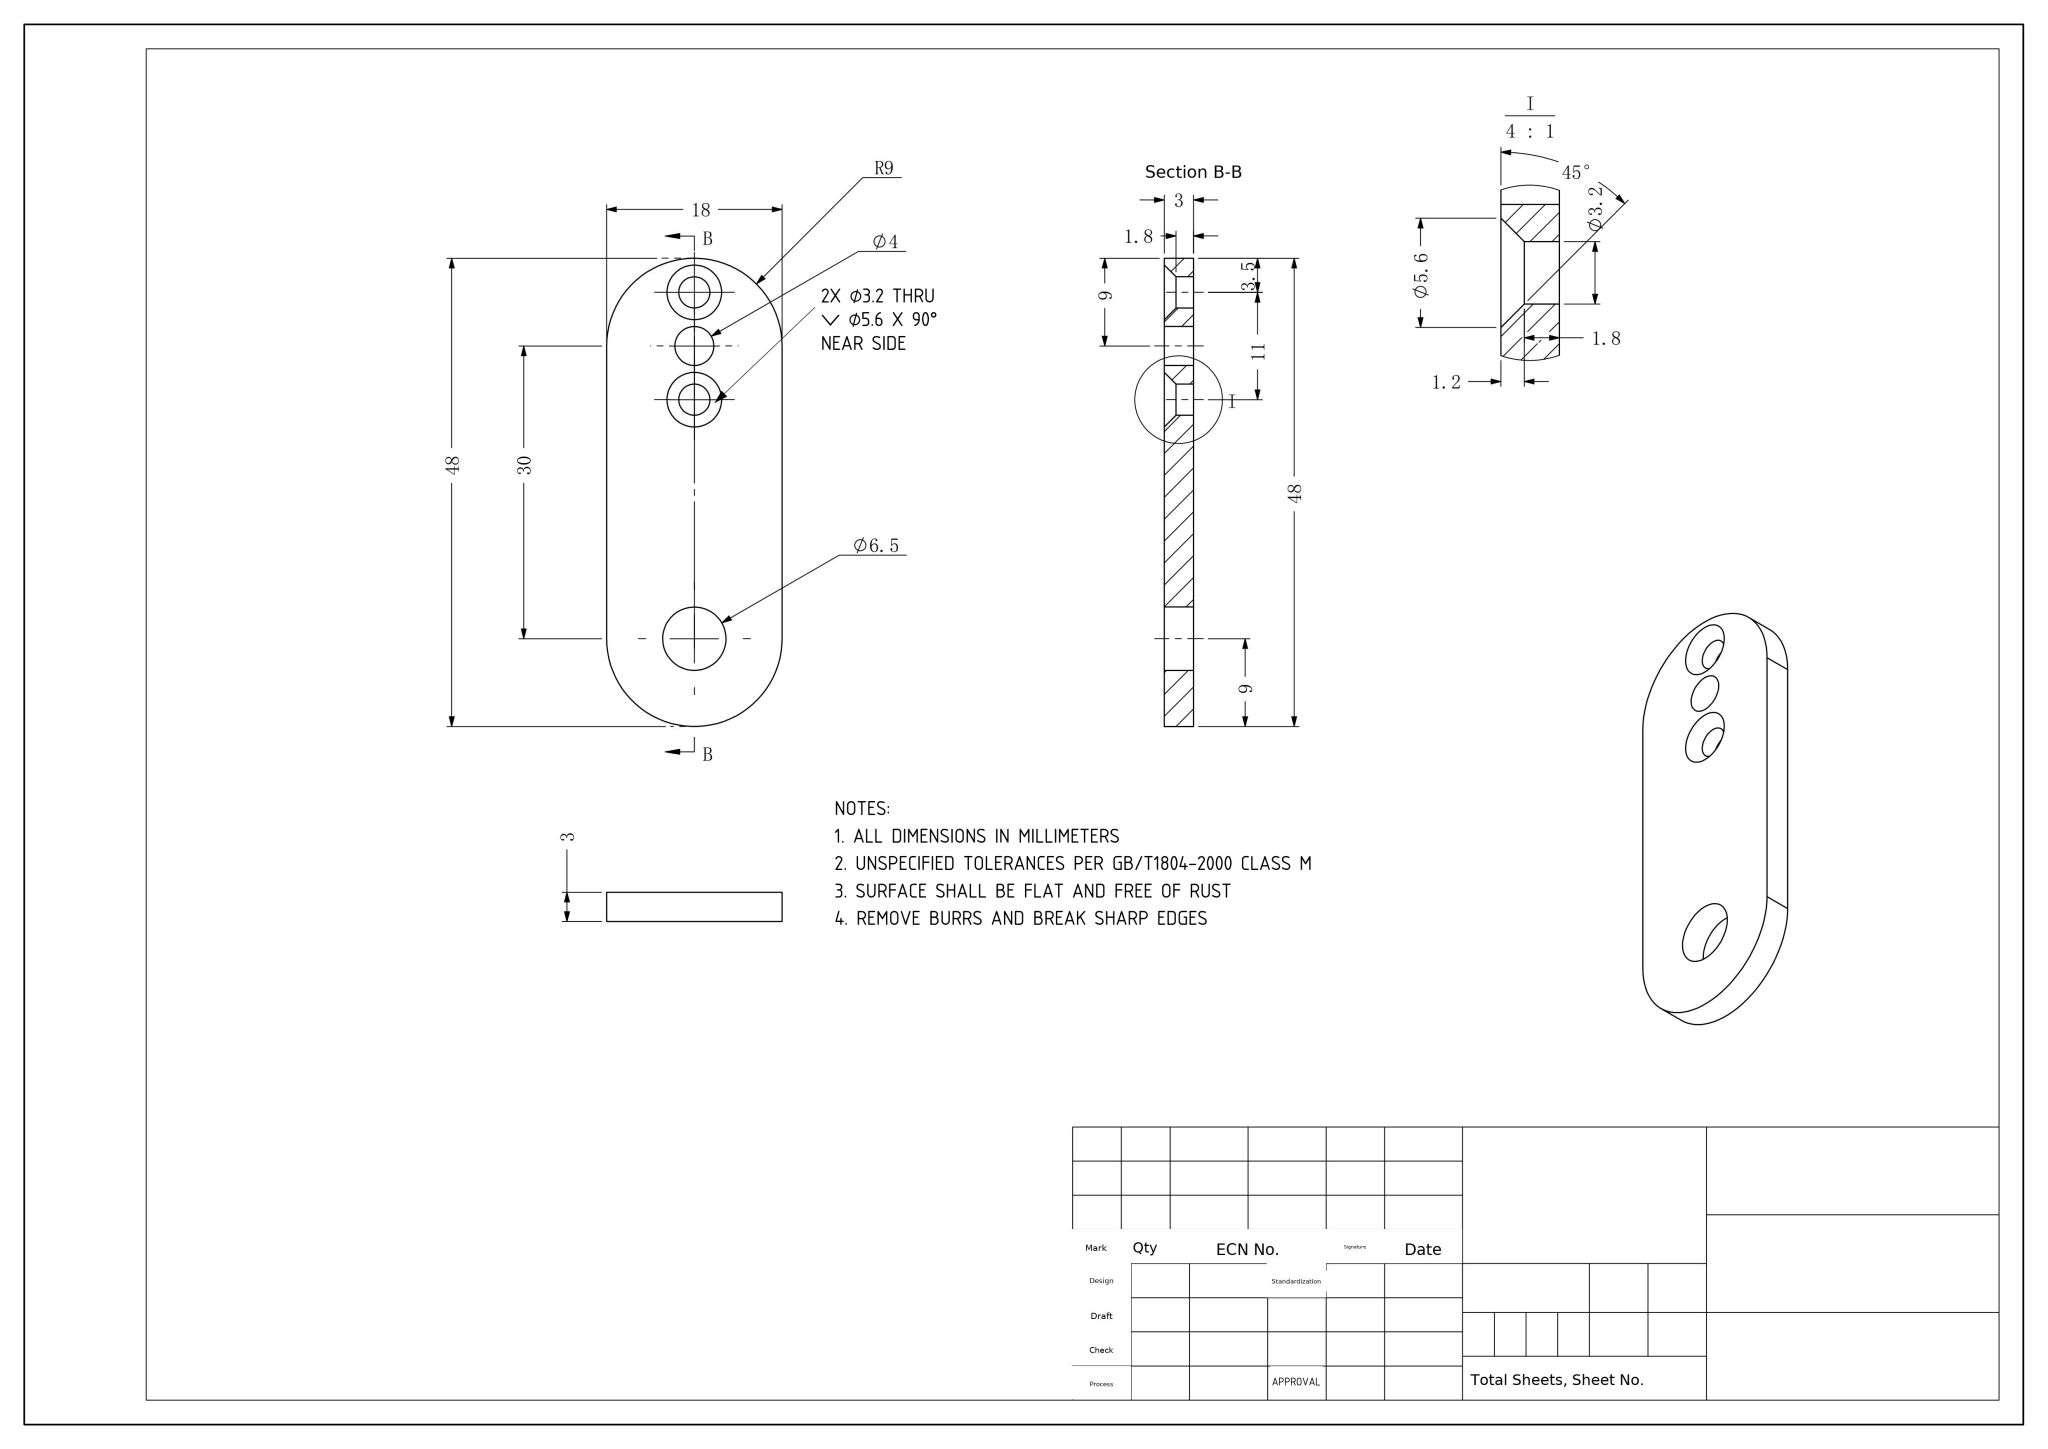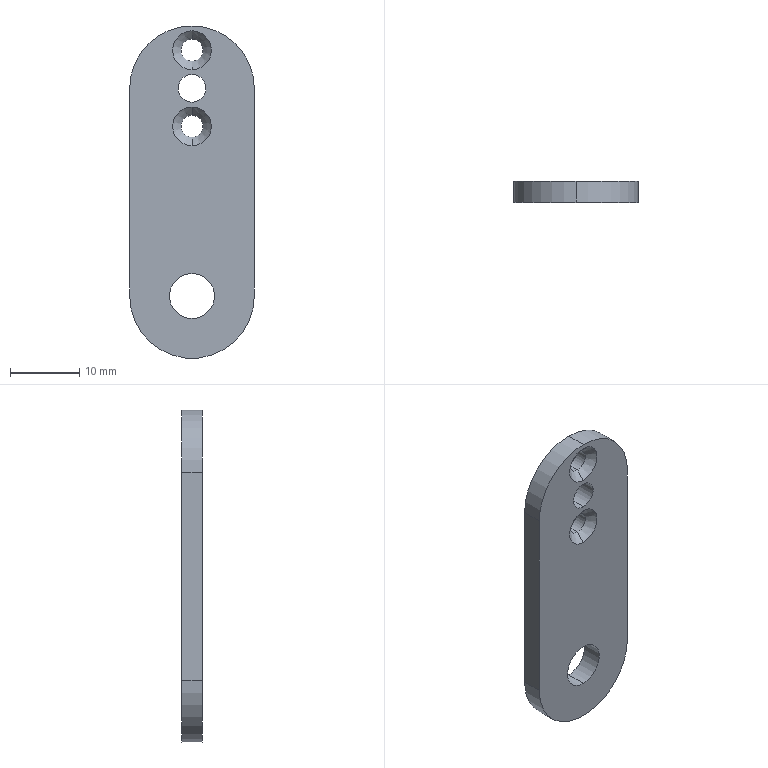Part | NX | mm | Rounded Four-Bore Link Plate | 1 solid | 19 faces | box 18 x 3 x 48 mm | volume 2180 mm3 | cylinder 11 | cone 4 | plane 4 | commonest cylinder face diameters 3.2 x4 18 x3 6.5 x2 4 x2
STEP:
#1=COLOUR_RGB('',0.7529,0.7529,0.7529);
#2=FILL_AREA_STYLE_COLOUR('',#1);
#3=FILL_AREA_STYLE('',(#2));
#4=SURFACE_STYLE_FILL_AREA(#3);
#5=SURFACE_SIDE_STYLE('',(#4));
#6=SURFACE_STYLE_USAGE(.BOTH.,#5);
#7=PRESENTATION_STYLE_ASSIGNMENT((#6));
#8=CARTESIAN_POINT('',(1.,-0.3,21.1));
#9=VERTEX_POINT('',#8);
#10=CARTESIAN_POINT('',(1.,-0.3,17.9));
#11=VERTEX_POINT('',#10);
#12=CARTESIAN_POINT('',(1.,-0.3,19.5));
#13=DIRECTION('',(0.,-1.,0.));
#14=DIRECTION('',(0.,0.,-1.));
#15=AXIS2_PLACEMENT_3D('',#12,#13,#14);
#16=CIRCLE('',#15,1.6);
#17=EDGE_CURVE('',#9,#11,#16,.T.);
#18=ORIENTED_EDGE('',*,*,#17,.F.);
#19=CARTESIAN_POINT('',(1.,-1.5,22.3));
#20=VERTEX_POINT('',#19);
#21=CARTESIAN_POINT('',(1.,-1.5,22.3));
#22=DIRECTION('',(0.,-0.7071,0.7071));
#23=VECTOR('',#22,1000.);
#24=LINE('',#21,#23);
#25=EDGE_CURVE('',#9,#20,#24,.T.);
#26=ORIENTED_EDGE('',*,*,#25,.T.);
#27=CARTESIAN_POINT('',(1.,-1.5,16.7));
#28=VERTEX_POINT('',#27);
#29=CARTESIAN_POINT('',(1.,-1.5,19.5));
#30=DIRECTION('',(0.,1.,0.));
#31=DIRECTION('',(0.,0.,-1.));
#32=AXIS2_PLACEMENT_3D('',#29,#30,#31);
#33=CIRCLE('',#32,2.8);
#34=EDGE_CURVE('',#28,#20,#33,.T.);
#35=ORIENTED_EDGE('',*,*,#34,.F.);
#36=CARTESIAN_POINT('',(1.,-1.5,16.7));
#37=DIRECTION('',(0.,-0.7071,-0.7071));
#38=VECTOR('',#37,1000.);
#39=LINE('',#36,#38);
#40=EDGE_CURVE('',#11,#28,#39,.T.);
#41=ORIENTED_EDGE('',*,*,#40,.F.);
#42=EDGE_LOOP('',(#18,#26,#35,#41));
#43=FACE_OUTER_BOUND('',#42,.T.);
#44=CARTESIAN_POINT('',(1.,-1.5,19.5));
#45=DIRECTION('',(0.,-1.,0.));
#46=DIRECTION('',(0.,0.,-1.));
#47=AXIS2_PLACEMENT_3D('',#44,#45,#46);
#48=CONICAL_SURFACE('',#47,2.8,0.7854);
#49=ADVANCED_FACE('',(#43),#48,.F.);
#50=CARTESIAN_POINT('',(1.,-0.3,10.1));
#51=VERTEX_POINT('',#50);
#52=CARTESIAN_POINT('',(1.,-0.3,6.9));
#53=VERTEX_POINT('',#52);
#54=CARTESIAN_POINT('',(1.,-0.3,8.5));
#55=DIRECTION('',(0.,-1.,0.));
#56=DIRECTION('',(0.,0.,-1.));
#57=AXIS2_PLACEMENT_3D('',#54,#55,#56);
#58=CIRCLE('',#57,1.6);
#59=EDGE_CURVE('',#51,#53,#58,.T.);
#60=ORIENTED_EDGE('',*,*,#59,.F.);
#61=CARTESIAN_POINT('',(1.,-1.5,11.3));
#62=VERTEX_POINT('',#61);
#63=CARTESIAN_POINT('',(1.,-0.3,10.1));
#64=DIRECTION('',(0.,-0.7071,0.7071));
#65=VECTOR('',#64,1000.);
#66=LINE('',#63,#65);
#67=EDGE_CURVE('',#51,#62,#66,.T.);
#68=ORIENTED_EDGE('',*,*,#67,.T.);
#69=CARTESIAN_POINT('',(1.,-1.5,5.7));
#70=VERTEX_POINT('',#69);
#71=CARTESIAN_POINT('',(1.,-1.5,8.5));
#72=DIRECTION('',(0.,1.,0.));
#73=DIRECTION('',(0.,0.,-1.));
#74=AXIS2_PLACEMENT_3D('',#71,#72,#73);
#75=CIRCLE('',#74,2.8);
#76=EDGE_CURVE('',#70,#62,#75,.T.);
#77=ORIENTED_EDGE('',*,*,#76,.F.);
#78=CARTESIAN_POINT('',(1.,-0.3,6.9));
#79=DIRECTION('',(0.,-0.7071,-0.7071));
#80=VECTOR('',#79,1000.);
#81=LINE('',#78,#80);
#82=EDGE_CURVE('',#53,#70,#81,.T.);
#83=ORIENTED_EDGE('',*,*,#82,.F.);
#84=EDGE_LOOP('',(#60,#68,#77,#83));
#85=FACE_OUTER_BOUND('',#84,.T.);
#86=CARTESIAN_POINT('',(1.,-0.3,8.5));
#87=DIRECTION('',(0.,-1.,0.));
#88=DIRECTION('',(0.,0.,-1.));
#89=AXIS2_PLACEMENT_3D('',#86,#87,#88);
#90=CONICAL_SURFACE('',#89,1.6,0.7854);
#91=ADVANCED_FACE('',(#85),#90,.F.);
#92=CARTESIAN_POINT('',(1.,1.5,17.9));
#93=VERTEX_POINT('',#92);
#94=CARTESIAN_POINT('',(1.,1.5,21.1));
#95=VERTEX_POINT('',#94);
#96=CARTESIAN_POINT('',(1.,1.5,19.5));
#97=DIRECTION('',(0.,1.,0.));
#98=DIRECTION('',(0.,0.,-1.));
#99=AXIS2_PLACEMENT_3D('',#96,#97,#98);
#100=CIRCLE('',#99,1.6);
#101=EDGE_CURVE('',#93,#95,#100,.T.);
#102=ORIENTED_EDGE('',*,*,#101,.T.);
#103=CARTESIAN_POINT('',(1.,78.5,21.1));
#104=DIRECTION('',(0.,-1.,0.));
#105=VECTOR('',#104,1000.);
#106=LINE('',#103,#105);
#107=EDGE_CURVE('',#95,#9,#106,.T.);
#108=ORIENTED_EDGE('',*,*,#107,.T.);
#109=ORIENTED_EDGE('',*,*,#17,.T.);
#110=CARTESIAN_POINT('',(1.,78.5,17.9));
#111=DIRECTION('',(0.,-1.,0.));
#112=VECTOR('',#111,1000.);
#113=LINE('',#110,#112);
#114=EDGE_CURVE('',#93,#11,#113,.T.);
#115=ORIENTED_EDGE('',*,*,#114,.F.);
#116=EDGE_LOOP('',(#102,#108,#109,#115));
#117=FACE_OUTER_BOUND('',#116,.T.);
#118=CARTESIAN_POINT('',(1.,78.5,19.5));
#119=DIRECTION('',(0.,-1.,0.));
#120=DIRECTION('',(0.,0.,-1.));
#121=AXIS2_PLACEMENT_3D('',#118,#119,#120);
#122=CYLINDRICAL_SURFACE('',#121,1.6);
#123=ADVANCED_FACE('',(#117),#122,.F.);
#124=CARTESIAN_POINT('',(1.,1.5,10.1));
#125=VERTEX_POINT('',#124);
#126=CARTESIAN_POINT('',(1.,1.5,6.9));
#127=VERTEX_POINT('',#126);
#128=CARTESIAN_POINT('',(1.,1.5,8.5));
#129=DIRECTION('',(0.,-1.,0.));
#130=DIRECTION('',(0.,0.,-1.));
#131=AXIS2_PLACEMENT_3D('',#128,#129,#130);
#132=CIRCLE('',#131,1.6);
#133=EDGE_CURVE('',#125,#127,#132,.T.);
#134=ORIENTED_EDGE('',*,*,#133,.F.);
#135=CARTESIAN_POINT('',(1.,78.5,10.1));
#136=DIRECTION('',(0.,-1.,0.));
#137=VECTOR('',#136,1000.);
#138=LINE('',#135,#137);
#139=EDGE_CURVE('',#125,#51,#138,.T.);
#140=ORIENTED_EDGE('',*,*,#139,.T.);
#141=ORIENTED_EDGE('',*,*,#59,.T.);
#142=CARTESIAN_POINT('',(1.,78.5,6.9));
#143=DIRECTION('',(0.,-1.,0.));
#144=VECTOR('',#143,1000.);
#145=LINE('',#142,#144);
#146=EDGE_CURVE('',#127,#53,#145,.T.);
#147=ORIENTED_EDGE('',*,*,#146,.F.);
#148=EDGE_LOOP('',(#134,#140,#141,#147));
#149=FACE_OUTER_BOUND('',#148,.T.);
#150=CARTESIAN_POINT('',(1.,78.5,8.5));
#151=DIRECTION('',(0.,-1.,0.));
#152=DIRECTION('',(0.,0.,-1.));
#153=AXIS2_PLACEMENT_3D('',#150,#151,#152);
#154=CYLINDRICAL_SURFACE('',#153,1.6);
#155=ADVANCED_FACE('',(#149),#154,.F.);
#156=CARTESIAN_POINT('',(1.,1.5,-19.25));
#157=VERTEX_POINT('',#156);
#158=CARTESIAN_POINT('',(1.,1.5,-12.75));
#159=VERTEX_POINT('',#158);
#160=CARTESIAN_POINT('',(1.,1.5,-16.));
#161=DIRECTION('',(0.,1.,0.));
#162=DIRECTION('',(0.,0.,-1.));
#163=AXIS2_PLACEMENT_3D('',#160,#161,#162);
#164=CIRCLE('',#163,3.25);
#165=EDGE_CURVE('',#157,#159,#164,.T.);
#166=ORIENTED_EDGE('',*,*,#165,.T.);
#167=CARTESIAN_POINT('',(1.,-1.5,-12.75));
#168=VERTEX_POINT('',#167);
#169=CARTESIAN_POINT('',(1.,49.852,-12.75));
#170=DIRECTION('',(0.,-1.,0.));
#171=VECTOR('',#170,1000.);
#172=LINE('',#169,#171);
#173=EDGE_CURVE('',#159,#168,#172,.T.);
#174=ORIENTED_EDGE('',*,*,#173,.T.);
#175=CARTESIAN_POINT('',(1.,-1.5,-19.25));
#176=VERTEX_POINT('',#175);
#177=CARTESIAN_POINT('',(1.,-1.5,-16.));
#178=DIRECTION('',(0.,1.,0.));
#179=DIRECTION('',(0.,0.,-1.));
#180=AXIS2_PLACEMENT_3D('',#177,#178,#179);
#181=CIRCLE('',#180,3.25);
#182=EDGE_CURVE('',#176,#168,#181,.T.);
#183=ORIENTED_EDGE('',*,*,#182,.F.);
#184=CARTESIAN_POINT('',(1.,49.852,-19.25));
#185=DIRECTION('',(0.,-1.,0.));
#186=VECTOR('',#185,1000.);
#187=LINE('',#184,#186);
#188=EDGE_CURVE('',#157,#176,#187,.T.);
#189=ORIENTED_EDGE('',*,*,#188,.F.);
#190=EDGE_LOOP('',(#166,#174,#183,#189));
#191=FACE_OUTER_BOUND('',#190,.T.);
#192=CARTESIAN_POINT('',(1.,49.852,-16.));
#193=DIRECTION('',(0.,-1.,0.));
#194=DIRECTION('',(0.,0.,-1.));
#195=AXIS2_PLACEMENT_3D('',#192,#193,#194);
#196=CYLINDRICAL_SURFACE('',#195,3.25);
#197=ADVANCED_FACE('',(#191),#196,.F.);
#198=CARTESIAN_POINT('',(1.,1.5,12.));
#199=VERTEX_POINT('',#198);
#200=CARTESIAN_POINT('',(1.,1.5,16.));
#201=VERTEX_POINT('',#200);
#202=CARTESIAN_POINT('',(1.,1.5,14.));
#203=DIRECTION('',(0.,1.,0.));
#204=DIRECTION('',(0.,0.,-1.));
#205=AXIS2_PLACEMENT_3D('',#202,#203,#204);
#206=CIRCLE('',#205,2.);
#207=EDGE_CURVE('',#199,#201,#206,.T.);
#208=ORIENTED_EDGE('',*,*,#207,.T.);
#209=CARTESIAN_POINT('',(1.,-1.5,16.));
#210=VERTEX_POINT('',#209);
#211=CARTESIAN_POINT('',(1.,106.5,16.));
#212=DIRECTION('',(0.,-1.,0.));
#213=VECTOR('',#212,1000.);
#214=LINE('',#211,#213);
#215=EDGE_CURVE('',#201,#210,#214,.T.);
#216=ORIENTED_EDGE('',*,*,#215,.T.);
#217=CARTESIAN_POINT('',(1.,-1.5,12.));
#218=VERTEX_POINT('',#217);
#219=CARTESIAN_POINT('',(1.,-1.5,14.));
#220=DIRECTION('',(0.,1.,0.));
#221=DIRECTION('',(0.,0.,1.));
#222=AXIS2_PLACEMENT_3D('',#219,#220,#221);
#223=CIRCLE('',#222,2.);
#224=EDGE_CURVE('',#218,#210,#223,.T.);
#225=ORIENTED_EDGE('',*,*,#224,.F.);
#226=CARTESIAN_POINT('',(1.,106.5,12.));
#227=DIRECTION('',(0.,-1.,0.));
#228=VECTOR('',#227,1000.);
#229=LINE('',#226,#228);
#230=EDGE_CURVE('',#199,#218,#229,.T.);
#231=ORIENTED_EDGE('',*,*,#230,.F.);
#232=EDGE_LOOP('',(#208,#216,#225,#231));
#233=FACE_OUTER_BOUND('',#232,.T.);
#234=CARTESIAN_POINT('',(1.,106.5,14.));
#235=DIRECTION('',(0.,-1.,0.));
#236=DIRECTION('',(0.,0.,-1.));
#237=AXIS2_PLACEMENT_3D('',#234,#235,#236);
#238=CYLINDRICAL_SURFACE('',#237,2.);
#239=ADVANCED_FACE('',(#233),#238,.F.);
#240=CARTESIAN_POINT('',(1.,-1.5,23.));
#241=VERTEX_POINT('',#240);
#242=CARTESIAN_POINT('',(-8.,-1.5,14.));
#243=VERTEX_POINT('',#242);
#244=CARTESIAN_POINT('',(1.,-1.5,14.));
#245=DIRECTION('',(0.,-1.,0.));
#246=DIRECTION('',(0.,0.,-1.));
#247=AXIS2_PLACEMENT_3D('',#244,#245,#246);
#248=CIRCLE('',#247,9.);
#249=EDGE_CURVE('',#241,#243,#248,.T.);
#250=ORIENTED_EDGE('',*,*,#249,.F.);
#251=CARTESIAN_POINT('',(1.,1.5,23.));
#252=VERTEX_POINT('',#251);
#253=CARTESIAN_POINT('',(1.,-1.5,23.));
#254=DIRECTION('',(0.,1.,0.));
#255=VECTOR('',#254,1000.);
#256=LINE('',#253,#255);
#257=EDGE_CURVE('',#241,#252,#256,.T.);
#258=ORIENTED_EDGE('',*,*,#257,.T.);
#259=CARTESIAN_POINT('',(-8.,1.5,14.));
#260=VERTEX_POINT('',#259);
#261=CARTESIAN_POINT('',(1.,1.5,14.));
#262=DIRECTION('',(0.,1.,0.));
#263=DIRECTION('',(0.,0.,-1.));
#264=AXIS2_PLACEMENT_3D('',#261,#262,#263);
#265=CIRCLE('',#264,9.);
#266=EDGE_CURVE('',#260,#252,#265,.T.);
#267=ORIENTED_EDGE('',*,*,#266,.F.);
#268=CARTESIAN_POINT('',(-8.,-1.5,14.));
#269=DIRECTION('',(0.,1.,0.));
#270=VECTOR('',#269,1000.);
#271=LINE('',#268,#270);
#272=EDGE_CURVE('',#243,#260,#271,.T.);
#273=ORIENTED_EDGE('',*,*,#272,.F.);
#274=EDGE_LOOP('',(#250,#258,#267,#273));
#275=FACE_OUTER_BOUND('',#274,.T.);
#276=CARTESIAN_POINT('',(1.,-1.5,14.));
#277=DIRECTION('',(0.,1.,0.));
#278=DIRECTION('',(0.,0.,1.));
#279=AXIS2_PLACEMENT_3D('',#276,#277,#278);
#280=CYLINDRICAL_SURFACE('',#279,9.);
#281=ADVANCED_FACE('',(#275),#280,.T.);
#282=ORIENTED_EDGE('',*,*,#76,.T.);
#283=CARTESIAN_POINT('',(1.,-1.5,8.5));
#284=DIRECTION('',(0.,1.,0.));
#285=DIRECTION('',(0.,0.,-1.));
#286=AXIS2_PLACEMENT_3D('',#283,#284,#285);
#287=CIRCLE('',#286,2.8);
#288=EDGE_CURVE('',#62,#70,#287,.T.);
#289=ORIENTED_EDGE('',*,*,#288,.T.);
#290=EDGE_LOOP('',(#282,#289));
#291=FACE_BOUND('',#290,.T.);
#292=ORIENTED_EDGE('',*,*,#34,.T.);
#293=CARTESIAN_POINT('',(1.,-1.5,19.5));
#294=DIRECTION('',(0.,1.,0.));
#295=DIRECTION('',(0.,0.,-1.));
#296=AXIS2_PLACEMENT_3D('',#293,#294,#295);
#297=CIRCLE('',#296,2.8);
#298=EDGE_CURVE('',#20,#28,#297,.T.);
#299=ORIENTED_EDGE('',*,*,#298,.T.);
#300=EDGE_LOOP('',(#292,#299));
#301=FACE_BOUND('',#300,.T.);
#302=ORIENTED_EDGE('',*,*,#182,.T.);
#303=CARTESIAN_POINT('',(1.,-1.5,-16.));
#304=DIRECTION('',(0.,1.,0.));
#305=DIRECTION('',(0.,0.,-1.));
#306=AXIS2_PLACEMENT_3D('',#303,#304,#305);
#307=CIRCLE('',#306,3.25);
#308=EDGE_CURVE('',#168,#176,#307,.T.);
#309=ORIENTED_EDGE('',*,*,#308,.T.);
#310=EDGE_LOOP('',(#302,#309));
#311=FACE_BOUND('',#310,.T.);
#312=CARTESIAN_POINT('',(10.,-1.5,-16.));
#313=VERTEX_POINT('',#312);
#314=CARTESIAN_POINT('',(10.,-1.5,14.));
#315=VERTEX_POINT('',#314);
#316=CARTESIAN_POINT('',(10.,-1.5,-25.));
#317=DIRECTION('',(0.,0.,1.));
#318=VECTOR('',#317,1000.);
#319=LINE('',#316,#318);
#320=EDGE_CURVE('',#313,#315,#319,.T.);
#321=ORIENTED_EDGE('',*,*,#320,.T.);
#322=CARTESIAN_POINT('',(1.,-1.5,14.));
#323=DIRECTION('',(0.,-1.,0.));
#324=DIRECTION('',(0.,0.,-1.));
#325=AXIS2_PLACEMENT_3D('',#322,#323,#324);
#326=CIRCLE('',#325,9.);
#327=EDGE_CURVE('',#315,#241,#326,.T.);
#328=ORIENTED_EDGE('',*,*,#327,.T.);
#329=ORIENTED_EDGE('',*,*,#249,.T.);
#330=CARTESIAN_POINT('',(-8.,-1.5,-16.));
#331=VERTEX_POINT('',#330);
#332=CARTESIAN_POINT('',(-8.,-1.5,23.));
#333=DIRECTION('',(-0.,0.,-1.));
#334=VECTOR('',#333,1000.);
#335=LINE('',#332,#334);
#336=EDGE_CURVE('',#243,#331,#335,.T.);
#337=ORIENTED_EDGE('',*,*,#336,.T.);
#338=CARTESIAN_POINT('',(1.,-1.5,-16.));
#339=DIRECTION('',(0.,-1.,0.));
#340=DIRECTION('',(0.,0.,-1.));
#341=AXIS2_PLACEMENT_3D('',#338,#339,#340);
#342=CIRCLE('',#341,9.);
#343=EDGE_CURVE('',#331,#313,#342,.T.);
#344=ORIENTED_EDGE('',*,*,#343,.T.);
#345=EDGE_LOOP('',(#321,#328,#329,#337,#344));
#346=FACE_OUTER_BOUND('',#345,.T.);
#347=ORIENTED_EDGE('',*,*,#224,.T.);
#348=CARTESIAN_POINT('',(1.,-1.5,14.));
#349=DIRECTION('',(0.,1.,0.));
#350=DIRECTION('',(0.,0.,1.));
#351=AXIS2_PLACEMENT_3D('',#348,#349,#350);
#352=CIRCLE('',#351,2.);
#353=EDGE_CURVE('',#210,#218,#352,.T.);
#354=ORIENTED_EDGE('',*,*,#353,.T.);
#355=EDGE_LOOP('',(#347,#354));
#356=FACE_BOUND('',#355,.T.);
#357=CARTESIAN_POINT('',(-8.,-1.5,-25.));
#358=DIRECTION('',(0.,-1.,0.));
#359=DIRECTION('',(0.,0.,-1.));
#360=AXIS2_PLACEMENT_3D('',#357,#358,#359);
#361=PLANE('',#360);
#362=ADVANCED_FACE('',(#291,#301,#311,#346,#356),#361,.T.);
#363=ORIENTED_EDGE('',*,*,#165,.F.);
#364=CARTESIAN_POINT('',(1.,1.5,-16.));
#365=DIRECTION('',(0.,1.,0.));
#366=DIRECTION('',(0.,0.,-1.));
#367=AXIS2_PLACEMENT_3D('',#364,#365,#366);
#368=CIRCLE('',#367,3.25);
#369=EDGE_CURVE('',#159,#157,#368,.T.);
#370=ORIENTED_EDGE('',*,*,#369,.F.);
#371=EDGE_LOOP('',(#363,#370));
#372=FACE_BOUND('',#371,.T.);
#373=ORIENTED_EDGE('',*,*,#266,.T.);
#374=CARTESIAN_POINT('',(10.,1.5,14.));
#375=VERTEX_POINT('',#374);
#376=CARTESIAN_POINT('',(1.,1.5,14.));
#377=DIRECTION('',(0.,1.,0.));
#378=DIRECTION('',(0.,0.,-1.));
#379=AXIS2_PLACEMENT_3D('',#376,#377,#378);
#380=CIRCLE('',#379,9.);
#381=EDGE_CURVE('',#252,#375,#380,.T.);
#382=ORIENTED_EDGE('',*,*,#381,.T.);
#383=CARTESIAN_POINT('',(10.,1.5,-16.));
#384=VERTEX_POINT('',#383);
#385=CARTESIAN_POINT('',(10.,1.5,-25.));
#386=DIRECTION('',(0.,0.,1.));
#387=VECTOR('',#386,1000.);
#388=LINE('',#385,#387);
#389=EDGE_CURVE('',#384,#375,#388,.T.);
#390=ORIENTED_EDGE('',*,*,#389,.F.);
#391=CARTESIAN_POINT('',(-8.,1.5,-16.));
#392=VERTEX_POINT('',#391);
#393=CARTESIAN_POINT('',(1.,1.5,-16.));
#394=DIRECTION('',(0.,1.,0.));
#395=DIRECTION('',(0.,0.,-1.));
#396=AXIS2_PLACEMENT_3D('',#393,#394,#395);
#397=CIRCLE('',#396,9.);
#398=EDGE_CURVE('',#384,#392,#397,.T.);
#399=ORIENTED_EDGE('',*,*,#398,.T.);
#400=CARTESIAN_POINT('',(-8.,1.5,23.));
#401=DIRECTION('',(-0.,0.,-1.));
#402=VECTOR('',#401,1000.);
#403=LINE('',#400,#402);
#404=EDGE_CURVE('',#260,#392,#403,.T.);
#405=ORIENTED_EDGE('',*,*,#404,.F.);
#406=EDGE_LOOP('',(#373,#382,#390,#399,#405));
#407=FACE_OUTER_BOUND('',#406,.T.);
#408=ORIENTED_EDGE('',*,*,#207,.F.);
#409=CARTESIAN_POINT('',(1.,1.5,14.));
#410=DIRECTION('',(0.,1.,0.));
#411=DIRECTION('',(0.,0.,-1.));
#412=AXIS2_PLACEMENT_3D('',#409,#410,#411);
#413=CIRCLE('',#412,2.);
#414=EDGE_CURVE('',#201,#199,#413,.T.);
#415=ORIENTED_EDGE('',*,*,#414,.F.);
#416=EDGE_LOOP('',(#408,#415));
#417=FACE_BOUND('',#416,.T.);
#418=CARTESIAN_POINT('',(1.,1.5,8.5));
#419=DIRECTION('',(0.,-1.,0.));
#420=DIRECTION('',(0.,0.,-1.));
#421=AXIS2_PLACEMENT_3D('',#418,#419,#420);
#422=CIRCLE('',#421,1.6);
#423=EDGE_CURVE('',#127,#125,#422,.T.);
#424=ORIENTED_EDGE('',*,*,#423,.T.);
#425=ORIENTED_EDGE('',*,*,#133,.T.);
#426=EDGE_LOOP('',(#424,#425));
#427=FACE_BOUND('',#426,.T.);
#428=ORIENTED_EDGE('',*,*,#101,.F.);
#429=CARTESIAN_POINT('',(1.,1.5,19.5));
#430=DIRECTION('',(0.,1.,0.));
#431=DIRECTION('',(0.,0.,-1.));
#432=AXIS2_PLACEMENT_3D('',#429,#430,#431);
#433=CIRCLE('',#432,1.6);
#434=EDGE_CURVE('',#95,#93,#433,.T.);
#435=ORIENTED_EDGE('',*,*,#434,.F.);
#436=EDGE_LOOP('',(#428,#435));
#437=FACE_BOUND('',#436,.T.);
#438=CARTESIAN_POINT('',(-8.,1.5,-25.));
#439=DIRECTION('',(0.,-1.,0.));
#440=DIRECTION('',(0.,0.,-1.));
#441=AXIS2_PLACEMENT_3D('',#438,#439,#440);
#442=PLANE('',#441);
#443=ADVANCED_FACE('',(#372,#407,#417,#427,#437),#442,.F.);
#444=ORIENTED_EDGE('',*,*,#404,.T.);
#445=CARTESIAN_POINT('',(-8.,-1.5,-16.));
#446=DIRECTION('',(0.,-1.,0.));
#447=VECTOR('',#446,1000.);
#448=LINE('',#445,#447);
#449=EDGE_CURVE('',#392,#331,#448,.T.);
#450=ORIENTED_EDGE('',*,*,#449,.T.);
#451=ORIENTED_EDGE('',*,*,#336,.F.);
#452=ORIENTED_EDGE('',*,*,#272,.T.);
#453=EDGE_LOOP('',(#444,#450,#451,#452));
#454=FACE_OUTER_BOUND('',#453,.T.);
#455=CARTESIAN_POINT('',(-8.,-1.5,23.));
#456=DIRECTION('',(1.,0.,-0.));
#457=DIRECTION('',(-0.,0.,-1.));
#458=AXIS2_PLACEMENT_3D('',#455,#456,#457);
#459=PLANE('',#458);
#460=ADVANCED_FACE('',(#454),#459,.F.);
#461=ORIENTED_EDGE('',*,*,#389,.T.);
#462=CARTESIAN_POINT('',(10.,-1.5,14.));
#463=DIRECTION('',(0.,-1.,0.));
#464=VECTOR('',#463,1000.);
#465=LINE('',#462,#464);
#466=EDGE_CURVE('',#375,#315,#465,.T.);
#467=ORIENTED_EDGE('',*,*,#466,.T.);
#468=ORIENTED_EDGE('',*,*,#320,.F.);
#469=CARTESIAN_POINT('',(10.,-1.5,-16.));
#470=DIRECTION('',(0.,1.,0.));
#471=VECTOR('',#470,1000.);
#472=LINE('',#469,#471);
#473=EDGE_CURVE('',#313,#384,#472,.T.);
#474=ORIENTED_EDGE('',*,*,#473,.T.);
#475=EDGE_LOOP('',(#461,#467,#468,#474));
#476=FACE_OUTER_BOUND('',#475,.T.);
#477=CARTESIAN_POINT('',(10.,-1.5,-25.));
#478=DIRECTION('',(-1.,0.,0.));
#479=DIRECTION('',(0.,0.,1.));
#480=AXIS2_PLACEMENT_3D('',#477,#478,#479);
#481=PLANE('',#480);
#482=ADVANCED_FACE('',(#476),#481,.F.);
#483=ORIENTED_EDGE('',*,*,#257,.F.);
#484=ORIENTED_EDGE('',*,*,#327,.F.);
#485=ORIENTED_EDGE('',*,*,#466,.F.);
#486=ORIENTED_EDGE('',*,*,#381,.F.);
#487=EDGE_LOOP('',(#483,#484,#485,#486));
#488=FACE_OUTER_BOUND('',#487,.T.);
#489=CARTESIAN_POINT('',(1.,-1.5,14.));
#490=DIRECTION('',(0.,1.,0.));
#491=DIRECTION('',(0.,0.,1.));
#492=AXIS2_PLACEMENT_3D('',#489,#490,#491);
#493=CYLINDRICAL_SURFACE('',#492,9.);
#494=ADVANCED_FACE('',(#488),#493,.T.);
#495=ORIENTED_EDGE('',*,*,#343,.F.);
#496=ORIENTED_EDGE('',*,*,#449,.F.);
#497=ORIENTED_EDGE('',*,*,#398,.F.);
#498=ORIENTED_EDGE('',*,*,#473,.F.);
#499=EDGE_LOOP('',(#495,#496,#497,#498));
#500=FACE_OUTER_BOUND('',#499,.T.);
#501=CARTESIAN_POINT('',(1.,-1.5,-16.));
#502=DIRECTION('',(0.,1.,0.));
#503=DIRECTION('',(0.,0.,1.));
#504=AXIS2_PLACEMENT_3D('',#501,#502,#503);
#505=CYLINDRICAL_SURFACE('',#504,9.);
#506=ADVANCED_FACE('',(#500),#505,.T.);
#507=ORIENTED_EDGE('',*,*,#215,.F.);
#508=ORIENTED_EDGE('',*,*,#414,.T.);
#509=ORIENTED_EDGE('',*,*,#230,.T.);
#510=ORIENTED_EDGE('',*,*,#353,.F.);
#511=EDGE_LOOP('',(#507,#508,#509,#510));
#512=FACE_OUTER_BOUND('',#511,.T.);
#513=CARTESIAN_POINT('',(1.,106.5,14.));
#514=DIRECTION('',(0.,-1.,0.));
#515=DIRECTION('',(0.,0.,-1.));
#516=AXIS2_PLACEMENT_3D('',#513,#514,#515);
#517=CYLINDRICAL_SURFACE('',#516,2.);
#518=ADVANCED_FACE('',(#512),#517,.F.);
#519=ORIENTED_EDGE('',*,*,#173,.F.);
#520=ORIENTED_EDGE('',*,*,#369,.T.);
#521=ORIENTED_EDGE('',*,*,#188,.T.);
#522=ORIENTED_EDGE('',*,*,#308,.F.);
#523=EDGE_LOOP('',(#519,#520,#521,#522));
#524=FACE_OUTER_BOUND('',#523,.T.);
#525=CARTESIAN_POINT('',(1.,49.852,-16.));
#526=DIRECTION('',(0.,-1.,0.));
#527=DIRECTION('',(0.,0.,-1.));
#528=AXIS2_PLACEMENT_3D('',#525,#526,#527);
#529=CYLINDRICAL_SURFACE('',#528,3.25);
#530=ADVANCED_FACE('',(#524),#529,.F.);
#531=ORIENTED_EDGE('',*,*,#139,.F.);
#532=ORIENTED_EDGE('',*,*,#423,.F.);
#533=ORIENTED_EDGE('',*,*,#146,.T.);
#534=CARTESIAN_POINT('',(1.,-0.3,8.5));
#535=DIRECTION('',(0.,-1.,0.));
#536=DIRECTION('',(0.,0.,-1.));
#537=AXIS2_PLACEMENT_3D('',#534,#535,#536);
#538=CIRCLE('',#537,1.6);
#539=EDGE_CURVE('',#53,#51,#538,.T.);
#540=ORIENTED_EDGE('',*,*,#539,.T.);
#541=EDGE_LOOP('',(#531,#532,#533,#540));
#542=FACE_OUTER_BOUND('',#541,.T.);
#543=CARTESIAN_POINT('',(1.,78.5,8.5));
#544=DIRECTION('',(0.,-1.,0.));
#545=DIRECTION('',(0.,0.,-1.));
#546=AXIS2_PLACEMENT_3D('',#543,#544,#545);
#547=CYLINDRICAL_SURFACE('',#546,1.6);
#548=ADVANCED_FACE('',(#542),#547,.F.);
#549=ORIENTED_EDGE('',*,*,#107,.F.);
#550=ORIENTED_EDGE('',*,*,#434,.T.);
#551=ORIENTED_EDGE('',*,*,#114,.T.);
#552=CARTESIAN_POINT('',(1.,-0.3,19.5));
#553=DIRECTION('',(0.,-1.,0.));
#554=DIRECTION('',(0.,0.,-1.));
#555=AXIS2_PLACEMENT_3D('',#552,#553,#554);
#556=CIRCLE('',#555,1.6);
#557=EDGE_CURVE('',#11,#9,#556,.T.);
#558=ORIENTED_EDGE('',*,*,#557,.T.);
#559=EDGE_LOOP('',(#549,#550,#551,#558));
#560=FACE_OUTER_BOUND('',#559,.T.);
#561=CARTESIAN_POINT('',(1.,78.5,19.5));
#562=DIRECTION('',(0.,-1.,0.));
#563=DIRECTION('',(0.,0.,-1.));
#564=AXIS2_PLACEMENT_3D('',#561,#562,#563);
#565=CYLINDRICAL_SURFACE('',#564,1.6);
#566=ADVANCED_FACE('',(#560),#565,.F.);
#567=ORIENTED_EDGE('',*,*,#67,.F.);
#568=ORIENTED_EDGE('',*,*,#539,.F.);
#569=ORIENTED_EDGE('',*,*,#82,.T.);
#570=ORIENTED_EDGE('',*,*,#288,.F.);
#571=EDGE_LOOP('',(#567,#568,#569,#570));
#572=FACE_OUTER_BOUND('',#571,.T.);
#573=CARTESIAN_POINT('',(1.,-0.3,8.5));
#574=DIRECTION('',(0.,-1.,0.));
#575=DIRECTION('',(0.,0.,-1.));
#576=AXIS2_PLACEMENT_3D('',#573,#574,#575);
#577=CONICAL_SURFACE('',#576,1.6,0.7854);
#578=ADVANCED_FACE('',(#572),#577,.F.);
#579=ORIENTED_EDGE('',*,*,#25,.F.);
#580=ORIENTED_EDGE('',*,*,#557,.F.);
#581=ORIENTED_EDGE('',*,*,#40,.T.);
#582=ORIENTED_EDGE('',*,*,#298,.F.);
#583=EDGE_LOOP('',(#579,#580,#581,#582));
#584=FACE_OUTER_BOUND('',#583,.T.);
#585=CARTESIAN_POINT('',(1.,-1.5,19.5));
#586=DIRECTION('',(0.,-1.,0.));
#587=DIRECTION('',(0.,0.,-1.));
#588=AXIS2_PLACEMENT_3D('',#585,#586,#587);
#589=CONICAL_SURFACE('',#588,2.8,0.7854);
#590=ADVANCED_FACE('',(#584),#589,.F.);
#591=CLOSED_SHELL('',(#49,#91,#123,#155,#197,#239,#281,#362,#443,#460,#482,#494,#506,#518,#530,#548,#566,#578,#590));
#592=MANIFOLD_SOLID_BREP('',#591);
#593=CARTESIAN_POINT('',(0.,0.,0.));
#594=DIRECTION('',(0.,0.,1.));
#595=DIRECTION('',(1.,0.,0.));
#596=AXIS2_PLACEMENT_3D('',#593,#594,#595);
#597=(LENGTH_UNIT()NAMED_UNIT(*)SI_UNIT(.MILLI.,.METRE.));
#598=UNCERTAINTY_MEASURE_WITH_UNIT(LENGTH_MEASURE(0.00001),#597,'','');
#599=(NAMED_UNIT(*)PLANE_ANGLE_UNIT()SI_UNIT($,.RADIAN.));
#600=(NAMED_UNIT(*)SI_UNIT($,.STERADIAN.)SOLID_ANGLE_UNIT());
#601=(GEOMETRIC_REPRESENTATION_CONTEXT(3)GLOBAL_UNCERTAINTY_ASSIGNED_CONTEXT((#598))GLOBAL_UNIT_ASSIGNED_CONTEXT((#597,#599,#600))REPRESENTATION_CONTEXT('',''));
#602=ADVANCED_BREP_SHAPE_REPRESENTATION('',(#592,#596),#601);
#603=STYLED_ITEM('',(#7),#602);
#604=(LENGTH_UNIT()NAMED_UNIT(*)SI_UNIT(.MILLI.,.METRE.));
#605=UNCERTAINTY_MEASURE_WITH_UNIT(LENGTH_MEASURE(0.00001),#604,'','');
#606=(NAMED_UNIT(*)PLANE_ANGLE_UNIT()SI_UNIT($,.RADIAN.));
#607=(NAMED_UNIT(*)SI_UNIT($,.STERADIAN.)SOLID_ANGLE_UNIT());
#608=(GEOMETRIC_REPRESENTATION_CONTEXT(3)GLOBAL_UNCERTAINTY_ASSIGNED_CONTEXT((#605))GLOBAL_UNIT_ASSIGNED_CONTEXT((#604,#606,#607))REPRESENTATION_CONTEXT('',''));
#609=MECHANICAL_DESIGN_GEOMETRIC_PRESENTATION_REPRESENTATION('',(#603),#608);
#610=COLOUR_RGB('',0.7529,0.7529,0.7529);
#611=FILL_AREA_STYLE_COLOUR('',#610);
#612=FILL_AREA_STYLE('',(#611));
#613=SURFACE_STYLE_FILL_AREA(#612);
#614=SURFACE_SIDE_STYLE('',(#613));
#615=SURFACE_STYLE_USAGE(.BOTH.,#614);
#616=PRESENTATION_STYLE_ASSIGNMENT((#615));
#617=STYLED_ITEM('',(#616),#592);
#618=(LENGTH_UNIT()NAMED_UNIT(*)SI_UNIT(.MILLI.,.METRE.));
#619=UNCERTAINTY_MEASURE_WITH_UNIT(LENGTH_MEASURE(0.00001),#618,'','');
#620=(NAMED_UNIT(*)PLANE_ANGLE_UNIT()SI_UNIT($,.RADIAN.));
#621=(NAMED_UNIT(*)SI_UNIT($,.STERADIAN.)SOLID_ANGLE_UNIT());
#622=(GEOMETRIC_REPRESENTATION_CONTEXT(3)GLOBAL_UNCERTAINTY_ASSIGNED_CONTEXT((#619))GLOBAL_UNIT_ASSIGNED_CONTEXT((#618,#620,#621))REPRESENTATION_CONTEXT('',''));
#623=MECHANICAL_DESIGN_GEOMETRIC_PRESENTATION_REPRESENTATION('',(#617),#622);
#624=PRESENTATION_LAYER_ASSIGNMENT('','',(#617));
#625=PRESENTATION_LAYER_ASSIGNMENT('','',(#603));